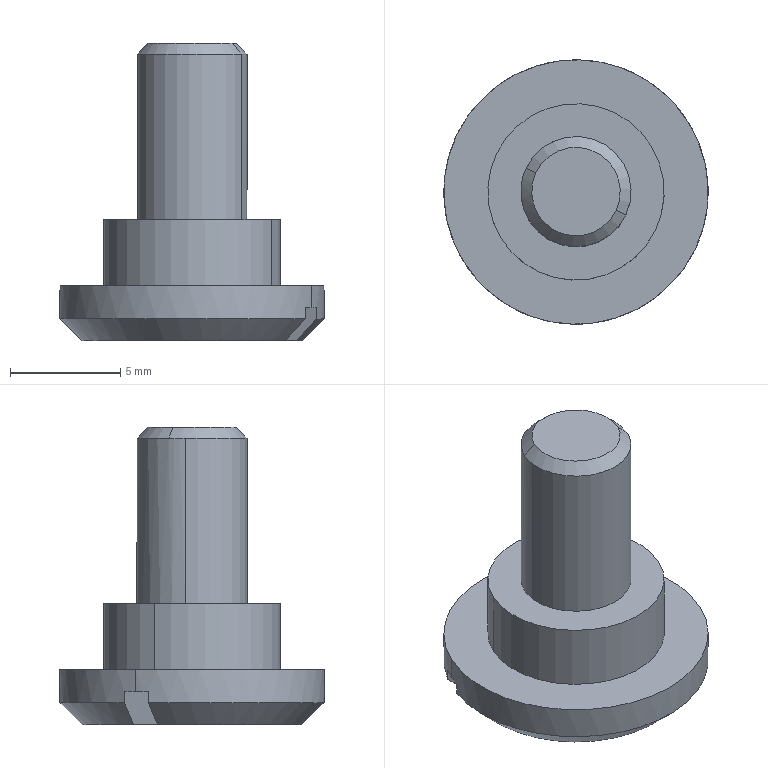Component | SolidWorks | StepScrewForFulcrumMJR06_D8_L3_A12_E2_5_F8-1 | 1 solid | 18 faces | box 12 x 12 x 13.5 mm | volume 551 mm3 | plane 8 | cylinder 6 | cone 4 | commonest cylinder face diameters 12 x2 8 x2 5 x2
STEP:
#1=COLOUR_RGB('',0.7922,0.8196,0.9333);
#2=FILL_AREA_STYLE_COLOUR('',#1);
#3=FILL_AREA_STYLE('',(#2));
#4=SURFACE_STYLE_FILL_AREA(#3);
#5=SURFACE_SIDE_STYLE('',(#4));
#6=SURFACE_STYLE_USAGE(.BOTH.,#5);
#7=PRESENTATION_STYLE_ASSIGNMENT((#6));
#8=CARTESIAN_POINT('',(-3.218,-0.3715,-1.319));
#9=VERTEX_POINT('',#8);
#10=CARTESIAN_POINT('',(-2.865,-0.5374,-1.319));
#11=VERTEX_POINT('',#10);
#12=CARTESIAN_POINT('',(-3.031,-0.4331,-1.319));
#13=DIRECTION('',(0.,0.,1.));
#14=DIRECTION('',(0.9055,-0.4244,0.));
#15=AXIS2_PLACEMENT_3D('',#12,#13,#14);
#16=CIRCLE('',#15,0.1969);
#17=EDGE_CURVE('',#9,#11,#16,.T.);
#18=ORIENTED_EDGE('',*,*,#17,.F.);
#19=CARTESIAN_POINT('',(-2.828,-0.5547,-1.319));
#20=DIRECTION('',(-0.9055,0.4244,-0.));
#21=VECTOR('',#20,39.37);
#22=LINE('',#19,#21);
#23=EDGE_CURVE('',#11,#9,#22,.T.);
#24=ORIENTED_EDGE('',*,*,#23,.F.);
#25=EDGE_LOOP('',(#18,#24));
#26=FACE_OUTER_BOUND('',#25,.T.);
#27=CARTESIAN_POINT('',(-3.031,-0.4331,-1.319));
#28=DIRECTION('',(0.,0.,1.));
#29=DIRECTION('',(0.9055,-0.4244,0.));
#30=AXIS2_PLACEMENT_3D('',#27,#28,#29);
#31=PLANE('',#30);
#32=ADVANCED_FACE('',(#26),#31,.F.);
#33=ORIENTED_EDGE('',*,*,#23,.T.);
#34=CARTESIAN_POINT('',(-3.254,-0.3547,-1.28));
#35=VERTEX_POINT('',#34);
#36=CARTESIAN_POINT('',(-3.254,-0.3547,-1.28));
#37=CARTESIAN_POINT('',(-3.242,-0.3603,-1.293));
#38=CARTESIAN_POINT('',(-3.23,-0.3659,-1.306));
#39=CARTESIAN_POINT('',(-3.218,-0.3715,-1.319));
#40=B_SPLINE_CURVE_WITH_KNOTS('',3,(#36,#37,#38,#39),.UNSPECIFIED.,.F.,.F.,(4,4),(0.,1.),.UNSPECIFIED.);
#41=EDGE_CURVE('',#35,#9,#40,.T.);
#42=ORIENTED_EDGE('',*,*,#41,.F.);
#43=CARTESIAN_POINT('',(-3.254,-0.3547,-1.26));
#44=VERTEX_POINT('',#43);
#45=CARTESIAN_POINT('',(-3.254,-0.3547,-1.22));
#46=DIRECTION('',(-0.,-0.,-1.));
#47=VECTOR('',#46,39.37);
#48=LINE('',#45,#47);
#49=EDGE_CURVE('',#44,#35,#48,.T.);
#50=ORIENTED_EDGE('',*,*,#49,.F.);
#51=CARTESIAN_POINT('',(-2.829,-0.5542,-1.26));
#52=VERTEX_POINT('',#51);
#53=CARTESIAN_POINT('',(-2.828,-0.5547,-1.26));
#54=DIRECTION('',(-0.9055,0.4244,-0.));
#55=VECTOR('',#54,39.37);
#56=LINE('',#53,#55);
#57=EDGE_CURVE('',#52,#44,#56,.T.);
#58=ORIENTED_EDGE('',*,*,#57,.F.);
#59=CARTESIAN_POINT('',(-2.829,-0.5542,-1.28));
#60=VERTEX_POINT('',#59);
#61=CARTESIAN_POINT('',(-2.829,-0.5542,-1.22));
#62=DIRECTION('',(0.,0.,1.));
#63=VECTOR('',#62,39.37);
#64=LINE('',#61,#63);
#65=EDGE_CURVE('',#60,#52,#64,.T.);
#66=ORIENTED_EDGE('',*,*,#65,.F.);
#67=CARTESIAN_POINT('',(-2.865,-0.5374,-1.319));
#68=CARTESIAN_POINT('',(-2.853,-0.543,-1.306));
#69=CARTESIAN_POINT('',(-2.841,-0.5486,-1.293));
#70=CARTESIAN_POINT('',(-2.829,-0.5542,-1.28));
#71=B_SPLINE_CURVE_WITH_KNOTS('',3,(#67,#68,#69,#70),.UNSPECIFIED.,.F.,.F.,(4,4),(0.,1.),.UNSPECIFIED.);
#72=EDGE_CURVE('',#11,#60,#71,.T.);
#73=ORIENTED_EDGE('',*,*,#72,.F.);
#74=EDGE_LOOP('',(#33,#42,#50,#58,#66,#73));
#75=FACE_OUTER_BOUND('',#74,.T.);
#76=CARTESIAN_POINT('',(-2.828,-0.5547,-1.26));
#77=DIRECTION('',(-0.4244,-0.9055,0.));
#78=DIRECTION('',(0.,0.,1.));
#79=AXIS2_PLACEMENT_3D('',#76,#77,#78);
#80=PLANE('',#79);
#81=ADVANCED_FACE('',(#75),#80,.F.);
#82=CARTESIAN_POINT('',(-3.031,-0.4331,-1.28));
#83=DIRECTION('',(0.,0.,1.));
#84=DIRECTION('',(0.9055,-0.4244,0.));
#85=AXIS2_PLACEMENT_3D('',#82,#83,#84);
#86=CIRCLE('',#85,0.2362);
#87=EDGE_CURVE('',#35,#60,#86,.T.);
#88=ORIENTED_EDGE('',*,*,#87,.F.);
#89=ORIENTED_EDGE('',*,*,#41,.T.);
#90=ORIENTED_EDGE('',*,*,#17,.T.);
#91=ORIENTED_EDGE('',*,*,#72,.T.);
#92=EDGE_LOOP('',(#88,#89,#90,#91));
#93=FACE_OUTER_BOUND('',#92,.T.);
#94=CARTESIAN_POINT('',(-3.031,-0.4331,-1.319));
#95=DIRECTION('',(0.,0.,1.));
#96=DIRECTION('',(0.4244,0.9055,0.));
#97=AXIS2_PLACEMENT_3D('',#94,#95,#96);
#98=CONICAL_SURFACE('',#97,0.1969,0.7854);
#99=ADVANCED_FACE('',(#93),#98,.T.);
#100=CARTESIAN_POINT('',(-3.245,-0.3328,-1.26));
#101=VERTEX_POINT('',#100);
#102=CARTESIAN_POINT('',(-3.245,-0.3328,-1.22));
#103=VERTEX_POINT('',#102);
#104=CARTESIAN_POINT('',(-3.245,-0.3328,-1.26));
#105=DIRECTION('',(0.,0.,1.));
#106=VECTOR('',#105,39.37);
#107=LINE('',#104,#106);
#108=EDGE_CURVE('',#101,#103,#107,.T.);
#109=ORIENTED_EDGE('',*,*,#108,.F.);
#110=CARTESIAN_POINT('',(-3.031,-0.4331,-1.26));
#111=DIRECTION('',(-0.,-0.,-1.));
#112=DIRECTION('',(-0.9055,0.4244,0.));
#113=AXIS2_PLACEMENT_3D('',#110,#111,#112);
#114=CIRCLE('',#113,0.2362);
#115=EDGE_CURVE('',#44,#101,#114,.T.);
#116=ORIENTED_EDGE('',*,*,#115,.F.);
#117=ORIENTED_EDGE('',*,*,#49,.T.);
#118=ORIENTED_EDGE('',*,*,#87,.T.);
#119=ORIENTED_EDGE('',*,*,#65,.T.);
#120=CARTESIAN_POINT('',(-2.818,-0.5333,-1.26));
#121=VERTEX_POINT('',#120);
#122=CARTESIAN_POINT('',(-3.031,-0.4331,-1.26));
#123=DIRECTION('',(-0.,-0.,-1.));
#124=DIRECTION('',(-0.9055,0.4244,0.));
#125=AXIS2_PLACEMENT_3D('',#122,#123,#124);
#126=CIRCLE('',#125,0.2362);
#127=EDGE_CURVE('',#121,#52,#126,.T.);
#128=ORIENTED_EDGE('',*,*,#127,.F.);
#129=CARTESIAN_POINT('',(-2.818,-0.5333,-1.22));
#130=VERTEX_POINT('',#129);
#131=CARTESIAN_POINT('',(-2.818,-0.5333,-1.26));
#132=DIRECTION('',(0.,0.,1.));
#133=VECTOR('',#132,39.37);
#134=LINE('',#131,#133);
#135=EDGE_CURVE('',#121,#130,#134,.T.);
#136=ORIENTED_EDGE('',*,*,#135,.T.);
#137=CARTESIAN_POINT('',(-3.031,-0.4331,-1.22));
#138=DIRECTION('',(0.,0.,1.));
#139=DIRECTION('',(0.9055,-0.4244,0.));
#140=AXIS2_PLACEMENT_3D('',#137,#138,#139);
#141=CIRCLE('',#140,0.2362);
#142=EDGE_CURVE('',#103,#130,#141,.T.);
#143=ORIENTED_EDGE('',*,*,#142,.F.);
#144=EDGE_LOOP('',(#109,#116,#117,#118,#119,#128,#136,#143));
#145=FACE_OUTER_BOUND('',#144,.T.);
#146=CARTESIAN_POINT('',(-3.031,-0.4331,-1.22));
#147=DIRECTION('',(0.,0.,1.));
#148=DIRECTION('',(0.4244,0.9055,0.));
#149=AXIS2_PLACEMENT_3D('',#146,#147,#148);
#150=CYLINDRICAL_SURFACE('',#149,0.2362);
#151=ADVANCED_FACE('',(#145),#150,.T.);
#152=CARTESIAN_POINT('',(-3.174,-0.3662,-1.22));
#153=VERTEX_POINT('',#152);
#154=CARTESIAN_POINT('',(-2.889,-0.4999,-1.22));
#155=VERTEX_POINT('',#154);
#156=CARTESIAN_POINT('',(-3.031,-0.4331,-1.22));
#157=DIRECTION('',(0.,0.,1.));
#158=DIRECTION('',(0.9055,-0.4244,0.));
#159=AXIS2_PLACEMENT_3D('',#156,#157,#158);
#160=CIRCLE('',#159,0.1575);
#161=EDGE_CURVE('',#153,#155,#160,.T.);
#162=ORIENTED_EDGE('',*,*,#161,.F.);
#163=CARTESIAN_POINT('',(-3.031,-0.4331,-1.22));
#164=DIRECTION('',(0.,0.,1.));
#165=DIRECTION('',(0.9055,-0.4244,0.));
#166=AXIS2_PLACEMENT_3D('',#163,#164,#165);
#167=CIRCLE('',#166,0.1575);
#168=EDGE_CURVE('',#155,#153,#167,.T.);
#169=ORIENTED_EDGE('',*,*,#168,.F.);
#170=EDGE_LOOP('',(#162,#169));
#171=FACE_BOUND('',#170,.T.);
#172=CARTESIAN_POINT('',(-3.031,-0.4331,-1.22));
#173=DIRECTION('',(0.,0.,1.));
#174=DIRECTION('',(0.9055,-0.4244,0.));
#175=AXIS2_PLACEMENT_3D('',#172,#173,#174);
#176=CIRCLE('',#175,0.2362);
#177=EDGE_CURVE('',#130,#103,#176,.T.);
#178=ORIENTED_EDGE('',*,*,#177,.T.);
#179=ORIENTED_EDGE('',*,*,#142,.T.);
#180=EDGE_LOOP('',(#178,#179));
#181=FACE_OUTER_BOUND('',#180,.T.);
#182=CARTESIAN_POINT('',(-2.931,-0.2192,-1.22));
#183=DIRECTION('',(-0.,-0.,-1.));
#184=DIRECTION('',(-0.9055,0.4244,-0.));
#185=AXIS2_PLACEMENT_3D('',#182,#183,#184);
#186=PLANE('',#185);
#187=ADVANCED_FACE('',(#171,#181),#186,.F.);
#188=ORIENTED_EDGE('',*,*,#108,.T.);
#189=ORIENTED_EDGE('',*,*,#177,.F.);
#190=ORIENTED_EDGE('',*,*,#135,.F.);
#191=CARTESIAN_POINT('',(-2.809,-0.5114,-1.26));
#192=VERTEX_POINT('',#191);
#193=CARTESIAN_POINT('',(-3.031,-0.4331,-1.26));
#194=DIRECTION('',(-0.,-0.,-1.));
#195=DIRECTION('',(-0.9055,0.4244,0.));
#196=AXIS2_PLACEMENT_3D('',#193,#194,#195);
#197=CIRCLE('',#196,0.2362);
#198=EDGE_CURVE('',#192,#121,#197,.T.);
#199=ORIENTED_EDGE('',*,*,#198,.F.);
#200=CARTESIAN_POINT('',(-2.809,-0.5114,-1.28));
#201=VERTEX_POINT('',#200);
#202=CARTESIAN_POINT('',(-2.809,-0.5114,-1.22));
#203=DIRECTION('',(-0.,-0.,-1.));
#204=VECTOR('',#203,39.37);
#205=LINE('',#202,#204);
#206=EDGE_CURVE('',#192,#201,#205,.T.);
#207=ORIENTED_EDGE('',*,*,#206,.T.);
#208=CARTESIAN_POINT('',(-3.234,-0.3119,-1.28));
#209=VERTEX_POINT('',#208);
#210=CARTESIAN_POINT('',(-3.031,-0.4331,-1.28));
#211=DIRECTION('',(0.,0.,1.));
#212=DIRECTION('',(0.9055,-0.4244,0.));
#213=AXIS2_PLACEMENT_3D('',#210,#211,#212);
#214=CIRCLE('',#213,0.2362);
#215=EDGE_CURVE('',#201,#209,#214,.T.);
#216=ORIENTED_EDGE('',*,*,#215,.T.);
#217=CARTESIAN_POINT('',(-3.234,-0.3119,-1.26));
#218=VERTEX_POINT('',#217);
#219=CARTESIAN_POINT('',(-3.234,-0.3119,-1.22));
#220=DIRECTION('',(0.,0.,1.));
#221=VECTOR('',#220,39.37);
#222=LINE('',#219,#221);
#223=EDGE_CURVE('',#209,#218,#222,.T.);
#224=ORIENTED_EDGE('',*,*,#223,.T.);
#225=CARTESIAN_POINT('',(-3.031,-0.4331,-1.26));
#226=DIRECTION('',(-0.,-0.,-1.));
#227=DIRECTION('',(-0.9055,0.4244,0.));
#228=AXIS2_PLACEMENT_3D('',#225,#226,#227);
#229=CIRCLE('',#228,0.2362);
#230=EDGE_CURVE('',#101,#218,#229,.T.);
#231=ORIENTED_EDGE('',*,*,#230,.F.);
#232=EDGE_LOOP('',(#188,#189,#190,#199,#207,#216,#224,#231));
#233=FACE_OUTER_BOUND('',#232,.T.);
#234=CARTESIAN_POINT('',(-3.031,-0.4331,-1.22));
#235=DIRECTION('',(0.,0.,1.));
#236=DIRECTION('',(-0.4244,-0.9055,0.));
#237=AXIS2_PLACEMENT_3D('',#234,#235,#236);
#238=CYLINDRICAL_SURFACE('',#237,0.2362);
#239=ADVANCED_FACE('',(#233),#238,.T.);
#240=CARTESIAN_POINT('',(-3.235,-0.3114,-1.26));
#241=DIRECTION('',(0.9055,-0.4244,0.));
#242=VECTOR('',#241,39.37);
#243=LINE('',#240,#242);
#244=EDGE_CURVE('',#218,#192,#243,.T.);
#245=ORIENTED_EDGE('',*,*,#244,.T.);
#246=ORIENTED_EDGE('',*,*,#198,.T.);
#247=ORIENTED_EDGE('',*,*,#127,.T.);
#248=ORIENTED_EDGE('',*,*,#57,.T.);
#249=ORIENTED_EDGE('',*,*,#115,.T.);
#250=ORIENTED_EDGE('',*,*,#230,.T.);
#251=EDGE_LOOP('',(#245,#246,#247,#248,#249,#250));
#252=FACE_OUTER_BOUND('',#251,.T.);
#253=CARTESIAN_POINT('',(-3.031,-0.4331,-1.26));
#254=DIRECTION('',(-0.,-0.,-1.));
#255=DIRECTION('',(-0.9055,0.4244,-0.));
#256=AXIS2_PLACEMENT_3D('',#253,#254,#255);
#257=PLANE('',#256);
#258=ADVANCED_FACE('',(#252),#257,.T.);
#259=CARTESIAN_POINT('',(-3.198,-0.3287,-1.319));
#260=VERTEX_POINT('',#259);
#261=CARTESIAN_POINT('',(-3.198,-0.3287,-1.319));
#262=CARTESIAN_POINT('',(-3.21,-0.3231,-1.306));
#263=CARTESIAN_POINT('',(-3.222,-0.3175,-1.293));
#264=CARTESIAN_POINT('',(-3.234,-0.3119,-1.28));
#265=B_SPLINE_CURVE_WITH_KNOTS('',3,(#261,#262,#263,#264),.UNSPECIFIED.,.F.,.F.,(4,4),(0.,1.),.UNSPECIFIED.);
#266=EDGE_CURVE('',#260,#209,#265,.T.);
#267=ORIENTED_EDGE('',*,*,#266,.F.);
#268=CARTESIAN_POINT('',(-2.845,-0.4946,-1.319));
#269=VERTEX_POINT('',#268);
#270=CARTESIAN_POINT('',(-3.235,-0.3114,-1.319));
#271=DIRECTION('',(0.9055,-0.4244,0.));
#272=VECTOR('',#271,39.37);
#273=LINE('',#270,#272);
#274=EDGE_CURVE('',#260,#269,#273,.T.);
#275=ORIENTED_EDGE('',*,*,#274,.T.);
#276=CARTESIAN_POINT('',(-2.809,-0.5114,-1.28));
#277=CARTESIAN_POINT('',(-2.821,-0.5058,-1.293));
#278=CARTESIAN_POINT('',(-2.833,-0.5002,-1.306));
#279=CARTESIAN_POINT('',(-2.845,-0.4946,-1.319));
#280=B_SPLINE_CURVE_WITH_KNOTS('',3,(#276,#277,#278,#279),.UNSPECIFIED.,.F.,.F.,(4,4),(0.,1.),.UNSPECIFIED.);
#281=EDGE_CURVE('',#201,#269,#280,.T.);
#282=ORIENTED_EDGE('',*,*,#281,.F.);
#283=ORIENTED_EDGE('',*,*,#206,.F.);
#284=ORIENTED_EDGE('',*,*,#244,.F.);
#285=ORIENTED_EDGE('',*,*,#223,.F.);
#286=EDGE_LOOP('',(#267,#275,#282,#283,#284,#285));
#287=FACE_OUTER_BOUND('',#286,.T.);
#288=CARTESIAN_POINT('',(-3.235,-0.3114,-1.26));
#289=DIRECTION('',(0.4244,0.9055,-0.));
#290=DIRECTION('',(-0.,-0.,-1.));
#291=AXIS2_PLACEMENT_3D('',#288,#289,#290);
#292=PLANE('',#291);
#293=ADVANCED_FACE('',(#287),#292,.F.);
#294=CARTESIAN_POINT('',(-3.031,-0.4331,-1.319));
#295=DIRECTION('',(0.,0.,1.));
#296=DIRECTION('',(0.9055,-0.4244,0.));
#297=AXIS2_PLACEMENT_3D('',#294,#295,#296);
#298=CIRCLE('',#297,0.1969);
#299=EDGE_CURVE('',#269,#260,#298,.T.);
#300=ORIENTED_EDGE('',*,*,#299,.T.);
#301=ORIENTED_EDGE('',*,*,#266,.T.);
#302=ORIENTED_EDGE('',*,*,#215,.F.);
#303=ORIENTED_EDGE('',*,*,#281,.T.);
#304=EDGE_LOOP('',(#300,#301,#302,#303));
#305=FACE_OUTER_BOUND('',#304,.T.);
#306=CARTESIAN_POINT('',(-3.031,-0.4331,-1.319));
#307=DIRECTION('',(0.,0.,1.));
#308=DIRECTION('',(-0.4244,-0.9055,0.));
#309=AXIS2_PLACEMENT_3D('',#306,#307,#308);
#310=CONICAL_SURFACE('',#309,0.1969,0.7854);
#311=ADVANCED_FACE('',(#305),#310,.T.);
#312=ORIENTED_EDGE('',*,*,#299,.F.);
#313=ORIENTED_EDGE('',*,*,#274,.F.);
#314=EDGE_LOOP('',(#312,#313));
#315=FACE_OUTER_BOUND('',#314,.T.);
#316=CARTESIAN_POINT('',(-3.031,-0.4331,-1.319));
#317=DIRECTION('',(0.,0.,1.));
#318=DIRECTION('',(0.9055,-0.4244,0.));
#319=AXIS2_PLACEMENT_3D('',#316,#317,#318);
#320=PLANE('',#319);
#321=ADVANCED_FACE('',(#315),#320,.F.);
#322=CARTESIAN_POINT('',(-3.174,-0.3662,-1.102));
#323=VERTEX_POINT('',#322);
#324=CARTESIAN_POINT('',(-3.174,-0.3662,-1.22));
#325=DIRECTION('',(0.,0.,1.));
#326=VECTOR('',#325,39.37);
#327=LINE('',#324,#326);
#328=EDGE_CURVE('',#153,#323,#327,.T.);
#329=ORIENTED_EDGE('',*,*,#328,.T.);
#330=CARTESIAN_POINT('',(-2.889,-0.4999,-1.102));
#331=VERTEX_POINT('',#330);
#332=CARTESIAN_POINT('',(-3.031,-0.4331,-1.102));
#333=DIRECTION('',(0.,0.,1.));
#334=DIRECTION('',(0.9055,-0.4244,0.));
#335=AXIS2_PLACEMENT_3D('',#332,#333,#334);
#336=CIRCLE('',#335,0.1575);
#337=EDGE_CURVE('',#331,#323,#336,.T.);
#338=ORIENTED_EDGE('',*,*,#337,.F.);
#339=CARTESIAN_POINT('',(-2.889,-0.4999,-1.22));
#340=DIRECTION('',(0.,0.,1.));
#341=VECTOR('',#340,39.37);
#342=LINE('',#339,#341);
#343=EDGE_CURVE('',#155,#331,#342,.T.);
#344=ORIENTED_EDGE('',*,*,#343,.F.);
#345=ORIENTED_EDGE('',*,*,#168,.T.);
#346=EDGE_LOOP('',(#329,#338,#344,#345));
#347=FACE_OUTER_BOUND('',#346,.T.);
#348=CARTESIAN_POINT('',(-3.031,-0.4331,-0.7874));
#349=DIRECTION('',(0.,0.,1.));
#350=DIRECTION('',(-0.4244,-0.9055,0.));
#351=AXIS2_PLACEMENT_3D('',#348,#349,#350);
#352=CYLINDRICAL_SURFACE('',#351,0.1575);
#353=ADVANCED_FACE('',(#347),#352,.T.);
#354=ORIENTED_EDGE('',*,*,#328,.F.);
#355=ORIENTED_EDGE('',*,*,#161,.T.);
#356=ORIENTED_EDGE('',*,*,#343,.T.);
#357=CARTESIAN_POINT('',(-3.031,-0.4331,-1.102));
#358=DIRECTION('',(0.,0.,1.));
#359=DIRECTION('',(0.9055,-0.4244,0.));
#360=AXIS2_PLACEMENT_3D('',#357,#358,#359);
#361=CIRCLE('',#360,0.1575);
#362=EDGE_CURVE('',#323,#331,#361,.T.);
#363=ORIENTED_EDGE('',*,*,#362,.F.);
#364=EDGE_LOOP('',(#354,#355,#356,#363));
#365=FACE_OUTER_BOUND('',#364,.T.);
#366=CARTESIAN_POINT('',(-3.031,-0.4331,-0.7874));
#367=DIRECTION('',(0.,0.,1.));
#368=DIRECTION('',(0.4244,0.9055,0.));
#369=AXIS2_PLACEMENT_3D('',#366,#367,#368);
#370=CYLINDRICAL_SURFACE('',#369,0.1575);
#371=ADVANCED_FACE('',(#365),#370,.T.);
#372=CARTESIAN_POINT('',(-3.129,-0.4209,-1.102));
#373=VERTEX_POINT('',#372);
#374=CARTESIAN_POINT('',(-2.942,-0.4748,-1.102));
#375=VERTEX_POINT('',#374);
#376=CARTESIAN_POINT('',(-3.031,-0.4331,-1.102));
#377=DIRECTION('',(0.,0.,1.));
#378=DIRECTION('',(0.9055,-0.4244,0.));
#379=AXIS2_PLACEMENT_3D('',#376,#377,#378);
#380=CIRCLE('',#379,0.09843);
#381=EDGE_CURVE('',#373,#375,#380,.T.);
#382=ORIENTED_EDGE('',*,*,#381,.F.);
#383=CARTESIAN_POINT('',(-3.031,-0.4331,-1.102));
#384=DIRECTION('',(0.,0.,1.));
#385=DIRECTION('',(0.9055,-0.4244,0.));
#386=AXIS2_PLACEMENT_3D('',#383,#384,#385);
#387=CIRCLE('',#386,0.09843);
#388=EDGE_CURVE('',#375,#373,#387,.T.);
#389=ORIENTED_EDGE('',*,*,#388,.F.);
#390=EDGE_LOOP('',(#382,#389));
#391=FACE_BOUND('',#390,.T.);
#392=ORIENTED_EDGE('',*,*,#337,.T.);
#393=ORIENTED_EDGE('',*,*,#362,.T.);
#394=EDGE_LOOP('',(#392,#393));
#395=FACE_OUTER_BOUND('',#394,.T.);
#396=CARTESIAN_POINT('',(-2.965,-0.2905,-1.102));
#397=DIRECTION('',(-0.,-0.,-1.));
#398=DIRECTION('',(-0.9055,0.4244,-0.));
#399=AXIS2_PLACEMENT_3D('',#396,#397,#398);
#400=PLANE('',#399);
#401=ADVANCED_FACE('',(#391,#395),#400,.F.);
#402=CARTESIAN_POINT('',(-3.129,-0.4209,-0.8067));
#403=VERTEX_POINT('',#402);
#404=CARTESIAN_POINT('',(-3.129,-0.4209,-1.102));
#405=DIRECTION('',(0.,0.,1.));
#406=VECTOR('',#405,39.37);
#407=LINE('',#404,#406);
#408=EDGE_CURVE('',#373,#403,#407,.T.);
#409=ORIENTED_EDGE('',*,*,#408,.T.);
#410=CARTESIAN_POINT('',(-3.121,-0.3913,-0.8067));
#411=VERTEX_POINT('',#410);
#412=CARTESIAN_POINT('',(-3.031,-0.4331,-0.8067));
#413=DIRECTION('',(0.,0.,1.));
#414=DIRECTION('',(0.9055,-0.4244,0.));
#415=AXIS2_PLACEMENT_3D('',#412,#413,#414);
#416=CIRCLE('',#415,0.09843);
#417=EDGE_CURVE('',#411,#403,#416,.T.);
#418=ORIENTED_EDGE('',*,*,#417,.F.);
#419=CARTESIAN_POINT('',(-2.942,-0.4748,-0.8067));
#420=VERTEX_POINT('',#419);
#421=CARTESIAN_POINT('',(-3.031,-0.4331,-0.8067));
#422=DIRECTION('',(0.,0.,1.));
#423=DIRECTION('',(0.9055,-0.4244,0.));
#424=AXIS2_PLACEMENT_3D('',#421,#422,#423);
#425=CIRCLE('',#424,0.09843);
#426=EDGE_CURVE('',#420,#411,#425,.T.);
#427=ORIENTED_EDGE('',*,*,#426,.F.);
#428=CARTESIAN_POINT('',(-2.942,-0.4748,-1.102));
#429=DIRECTION('',(0.,0.,1.));
#430=VECTOR('',#429,39.37);
#431=LINE('',#428,#430);
#432=EDGE_CURVE('',#375,#420,#431,.T.);
#433=ORIENTED_EDGE('',*,*,#432,.F.);
#434=ORIENTED_EDGE('',*,*,#388,.T.);
#435=EDGE_LOOP('',(#409,#418,#427,#433,#434));
#436=FACE_OUTER_BOUND('',#435,.T.);
#437=CARTESIAN_POINT('',(-3.031,-0.4331,-0.7874));
#438=DIRECTION('',(0.,0.,1.));
#439=DIRECTION('',(-0.2775,-0.9607,0.));
#440=AXIS2_PLACEMENT_3D('',#437,#438,#439);
#441=CYLINDRICAL_SURFACE('',#440,0.09843);
#442=ADVANCED_FACE('',(#436),#441,.T.);
#443=ORIENTED_EDGE('',*,*,#408,.F.);
#444=ORIENTED_EDGE('',*,*,#381,.T.);
#445=ORIENTED_EDGE('',*,*,#432,.T.);
#446=CARTESIAN_POINT('',(-3.031,-0.4331,-0.8067));
#447=DIRECTION('',(0.,0.,1.));
#448=DIRECTION('',(0.9055,-0.4244,0.));
#449=AXIS2_PLACEMENT_3D('',#446,#447,#448);
#450=CIRCLE('',#449,0.09843);
#451=EDGE_CURVE('',#403,#420,#450,.T.);
#452=ORIENTED_EDGE('',*,*,#451,.F.);
#453=EDGE_LOOP('',(#443,#444,#445,#452));
#454=FACE_OUTER_BOUND('',#453,.T.);
#455=CARTESIAN_POINT('',(-3.031,-0.4331,-0.7874));
#456=DIRECTION('',(0.,0.,1.));
#457=DIRECTION('',(0.2775,0.9607,0.));
#458=AXIS2_PLACEMENT_3D('',#455,#456,#457);
#459=CYLINDRICAL_SURFACE('',#458,0.09843);
#460=ADVANCED_FACE('',(#454),#459,.T.);
#461=CARTESIAN_POINT('',(-2.96,-0.4666,-0.7874));
#462=VERTEX_POINT('',#461);
#463=CARTESIAN_POINT('',(-2.96,-0.4666,-0.7874));
#464=DIRECTION('',(0.6403,-0.3001,-0.7071));
#465=VECTOR('',#464,39.37);
#466=LINE('',#463,#465);
#467=EDGE_CURVE('',#462,#420,#466,.T.);
#468=ORIENTED_EDGE('',*,*,#467,.F.);
#469=CARTESIAN_POINT('',(-3.103,-0.3995,-0.7874));
#470=VERTEX_POINT('',#469);
#471=CARTESIAN_POINT('',(-3.031,-0.4331,-0.7874));
#472=DIRECTION('',(0.,0.,1.));
#473=DIRECTION('',(0.9055,-0.4244,0.));
#474=AXIS2_PLACEMENT_3D('',#471,#472,#473);
#475=CIRCLE('',#474,0.07911);
#476=EDGE_CURVE('',#470,#462,#475,.T.);
#477=ORIENTED_EDGE('',*,*,#476,.F.);
#478=CARTESIAN_POINT('',(-3.103,-0.3995,-0.7874));
#479=DIRECTION('',(-0.6403,0.3001,-0.7071));
#480=VECTOR('',#479,39.37);
#481=LINE('',#478,#480);
#482=EDGE_CURVE('',#470,#411,#481,.T.);
#483=ORIENTED_EDGE('',*,*,#482,.T.);
#484=ORIENTED_EDGE('',*,*,#417,.T.);
#485=ORIENTED_EDGE('',*,*,#451,.T.);
#486=EDGE_LOOP('',(#468,#477,#483,#484,#485));
#487=FACE_OUTER_BOUND('',#486,.T.);
#488=CARTESIAN_POINT('',(-3.031,-0.4331,-0.8067));
#489=DIRECTION('',(-0.,-0.,-1.));
#490=DIRECTION('',(0.4244,0.9055,0.));
#491=AXIS2_PLACEMENT_3D('',#488,#489,#490);
#492=CONICAL_SURFACE('',#491,0.09843,0.7854);
#493=ADVANCED_FACE('',(#487),#492,.T.);
#494=ORIENTED_EDGE('',*,*,#467,.T.);
#495=ORIENTED_EDGE('',*,*,#426,.T.);
#496=ORIENTED_EDGE('',*,*,#482,.F.);
#497=CARTESIAN_POINT('',(-3.031,-0.4331,-0.7874));
#498=DIRECTION('',(0.,0.,1.));
#499=DIRECTION('',(0.9055,-0.4244,0.));
#500=AXIS2_PLACEMENT_3D('',#497,#498,#499);
#501=CIRCLE('',#500,0.07911);
#502=EDGE_CURVE('',#462,#470,#501,.T.);
#503=ORIENTED_EDGE('',*,*,#502,.F.);
#504=EDGE_LOOP('',(#494,#495,#496,#503));
#505=FACE_OUTER_BOUND('',#504,.T.);
#506=CARTESIAN_POINT('',(-3.031,-0.4331,-0.8067));
#507=DIRECTION('',(-0.,-0.,-1.));
#508=DIRECTION('',(-0.4244,-0.9055,0.));
#509=AXIS2_PLACEMENT_3D('',#506,#507,#508);
#510=CONICAL_SURFACE('',#509,0.09843,0.7854);
#511=ADVANCED_FACE('',(#505),#510,.T.);
#512=ORIENTED_EDGE('',*,*,#502,.T.);
#513=ORIENTED_EDGE('',*,*,#476,.T.);
#514=EDGE_LOOP('',(#512,#513));
#515=FACE_OUTER_BOUND('',#514,.T.);
#516=CARTESIAN_POINT('',(-2.998,-0.3614,-0.7874));
#517=DIRECTION('',(-0.,-0.,-1.));
#518=DIRECTION('',(-0.9055,0.4244,-0.));
#519=AXIS2_PLACEMENT_3D('',#516,#517,#518);
#520=PLANE('',#519);
#521=ADVANCED_FACE('',(#515),#520,.F.);
#522=CLOSED_SHELL('',(#32,#81,#99,#151,#187,#239,#258,#293,#311,#321,#353,#371,#401,#442,#460,#493,#511,#521));
#523=MANIFOLD_SOLID_BREP('',#522);
#524=STYLED_ITEM('',(#7),#523);
#525=(LENGTH_UNIT()NAMED_UNIT(*)SI_UNIT($,.METRE.));
#526=LENGTH_MEASURE_WITH_UNIT(LENGTH_MEASURE(0.0254),#525);
#527=DIMENSIONAL_EXPONENTS(1.,0.,0.,0.,0.,0.,0.);
#528=(CONVERSION_BASED_UNIT('',#526)LENGTH_UNIT()NAMED_UNIT(#527));
#529=UNCERTAINTY_MEASURE_WITH_UNIT(LENGTH_MEASURE(0.00001),#528,'','');
#530=(NAMED_UNIT(*)PLANE_ANGLE_UNIT()SI_UNIT($,.RADIAN.));
#531=(NAMED_UNIT(*)SI_UNIT($,.STERADIAN.)SOLID_ANGLE_UNIT());
#532=(GEOMETRIC_REPRESENTATION_CONTEXT(3)GLOBAL_UNCERTAINTY_ASSIGNED_CONTEXT((#529))GLOBAL_UNIT_ASSIGNED_CONTEXT((#528,#530,#531))REPRESENTATION_CONTEXT('',''));
#533=MECHANICAL_DESIGN_GEOMETRIC_PRESENTATION_REPRESENTATION('',(#524),#532);
#534=CARTESIAN_POINT('',(0.,0.,0.));
#535=DIRECTION('',(0.,0.,1.));
#536=DIRECTION('',(1.,0.,0.));
#537=AXIS2_PLACEMENT_3D('',#534,#535,#536);
#538=(LENGTH_UNIT()NAMED_UNIT(*)SI_UNIT($,.METRE.));
#539=LENGTH_MEASURE_WITH_UNIT(LENGTH_MEASURE(0.0254),#538);
#540=DIMENSIONAL_EXPONENTS(1.,0.,0.,0.,0.,0.,0.);
#541=(CONVERSION_BASED_UNIT('',#539)LENGTH_UNIT()NAMED_UNIT(#540));
#542=UNCERTAINTY_MEASURE_WITH_UNIT(LENGTH_MEASURE(0.00001),#541,'','');
#543=(NAMED_UNIT(*)PLANE_ANGLE_UNIT()SI_UNIT($,.RADIAN.));
#544=(NAMED_UNIT(*)SI_UNIT($,.STERADIAN.)SOLID_ANGLE_UNIT());
#545=(GEOMETRIC_REPRESENTATION_CONTEXT(3)GLOBAL_UNCERTAINTY_ASSIGNED_CONTEXT((#542))GLOBAL_UNIT_ASSIGNED_CONTEXT((#541,#543,#544))REPRESENTATION_CONTEXT('',''));
#546=ADVANCED_BREP_SHAPE_REPRESENTATION('',(#523,#537),#545);
#547=PRESENTATION_LAYER_ASSIGNMENT('','',(#524));